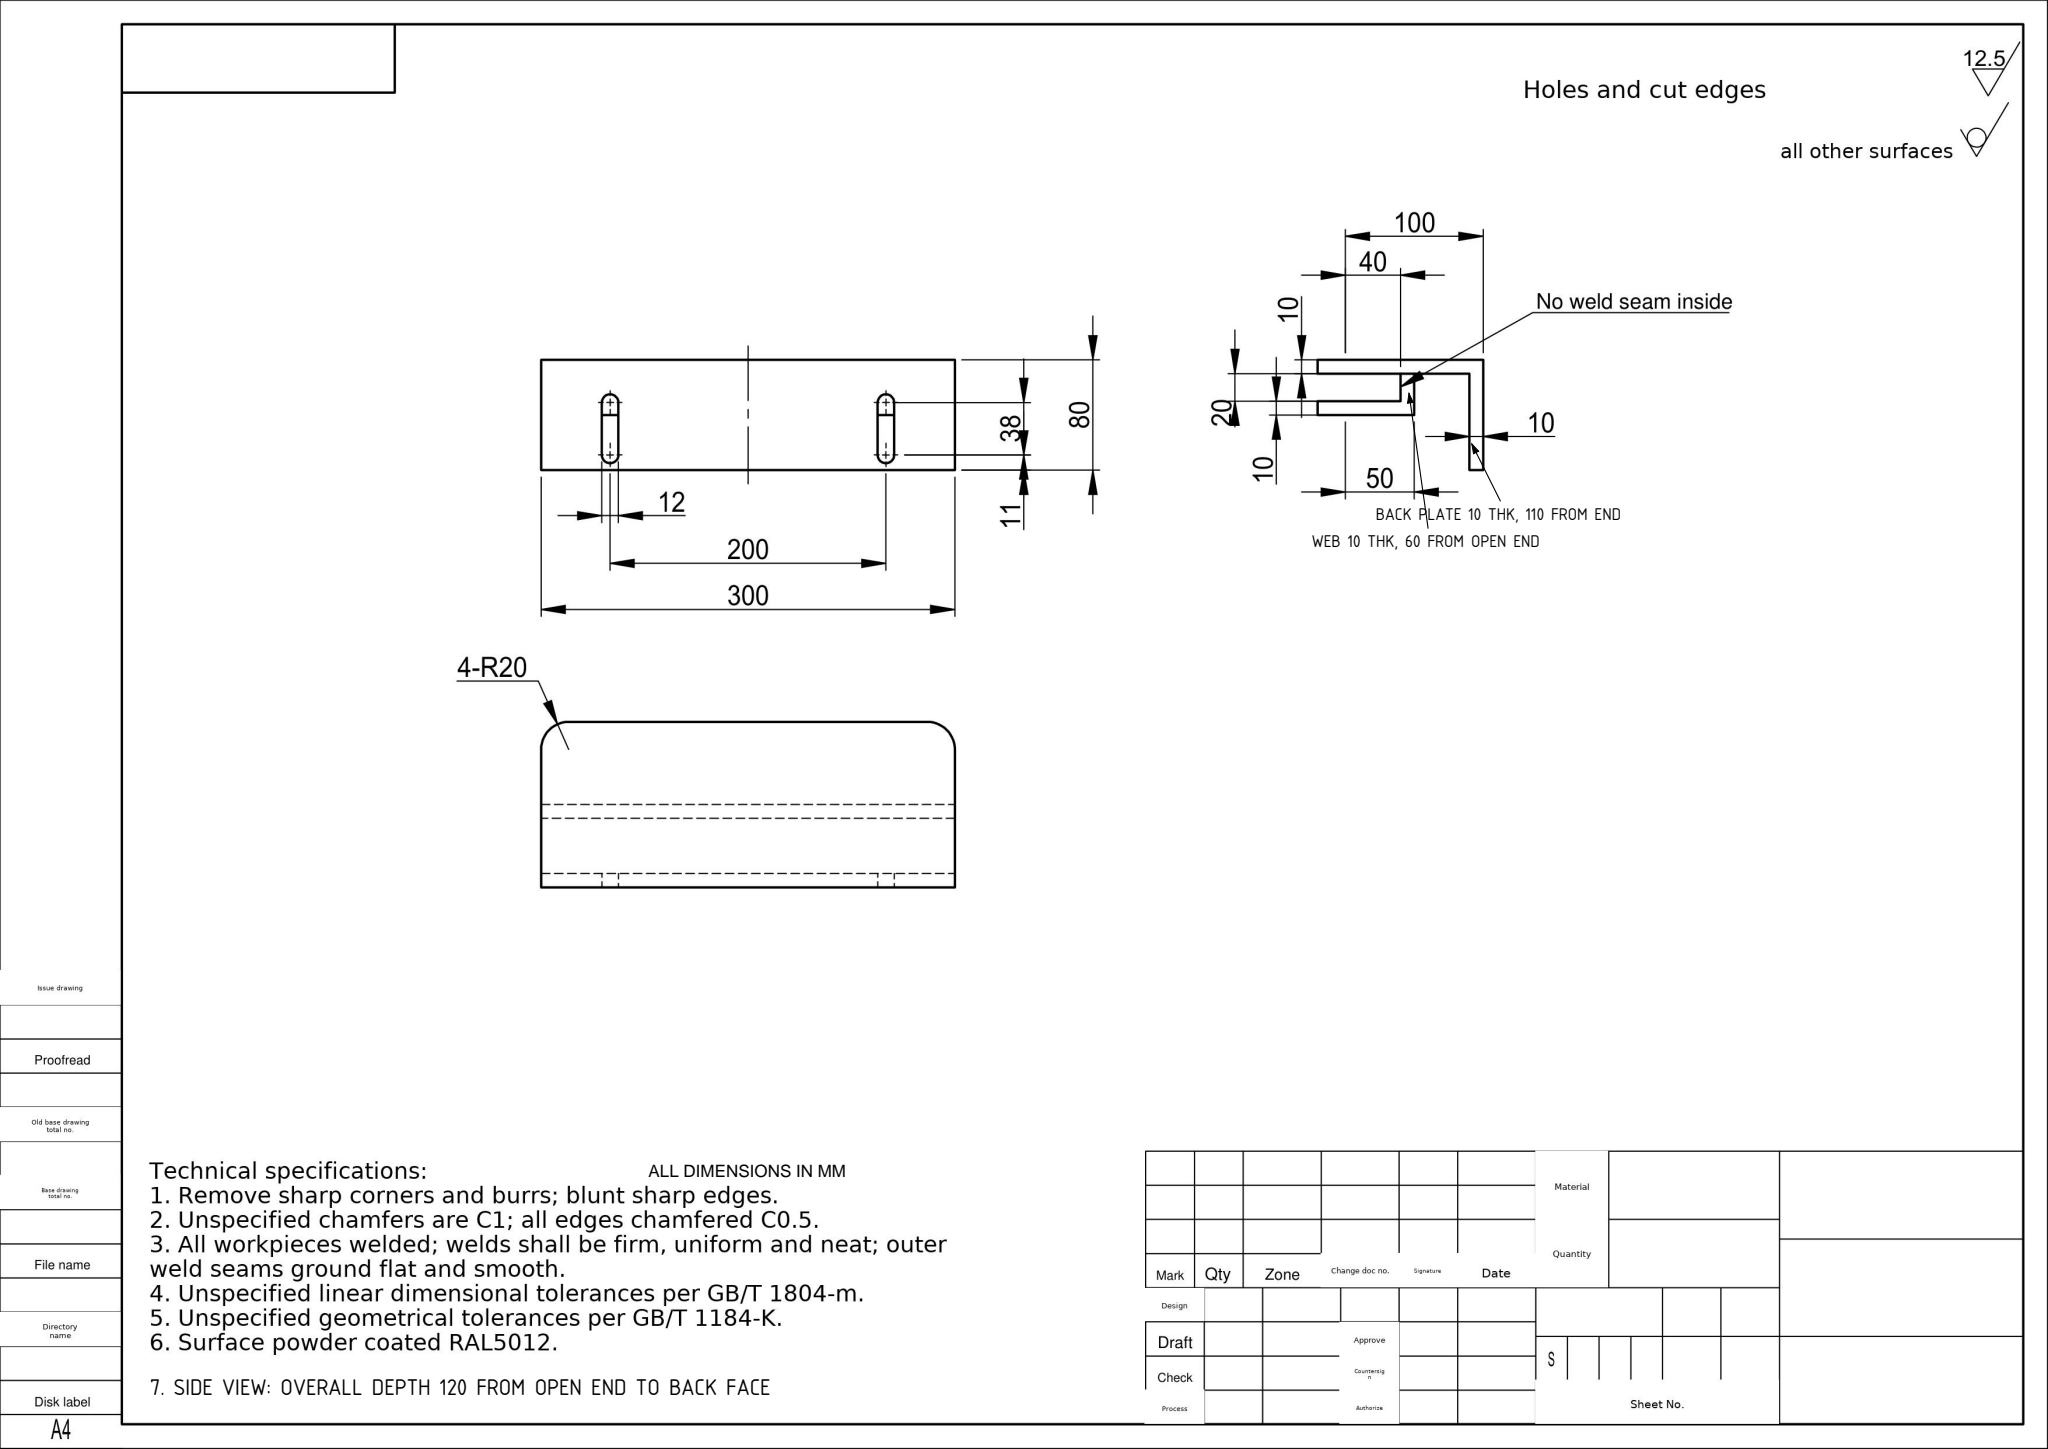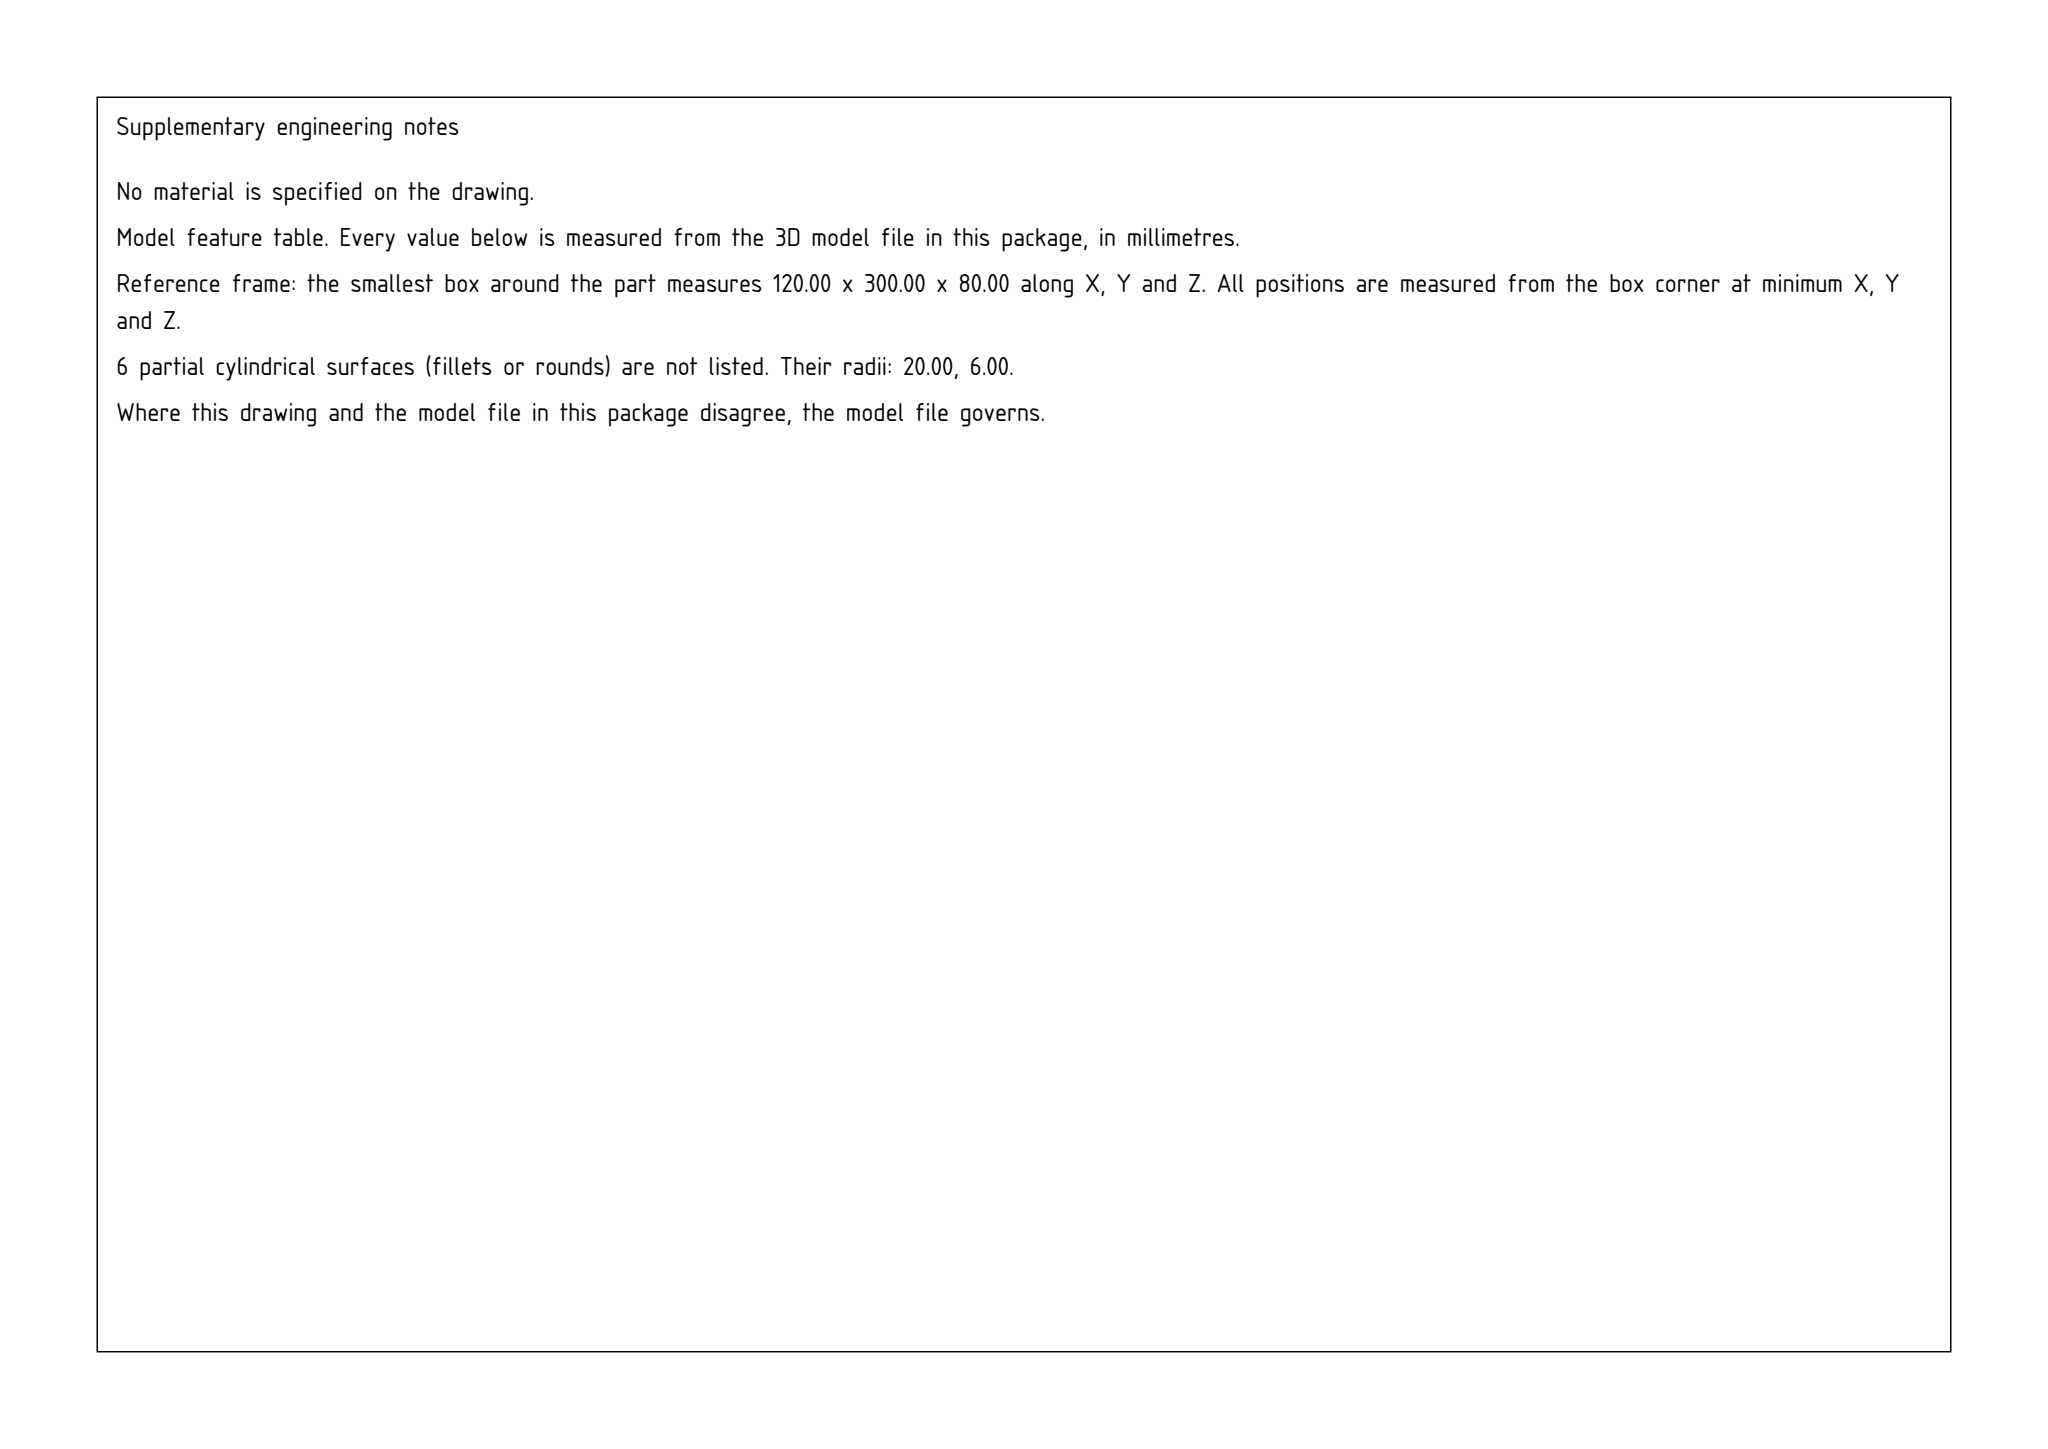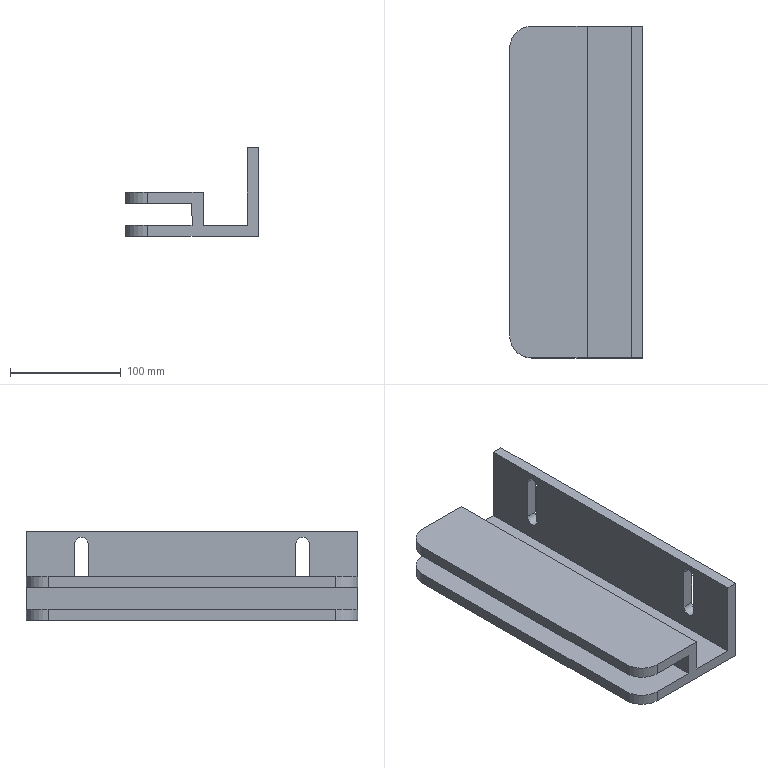Part | SolidWorks | mm | 1 solid | 28 faces | box 120 x 300 x 80 mm | volume 825184 mm3 | plane 18 | cylinder 10 | commonest cylinder face diameters 12 x6 40 x4
Drawing notes:
SIDE VIEW: OVERALL DEPTH 120 FROM OPEN END TO BACK FACE | from the solid: bbox_xyz x=120; planes x=0 (channel open end) and x=120 (back face)
BACK PLATE 10 THK: INNER FACE 110 FROM OPEN END | from the solid: plane x=110 (y 0-300, z 10-80) and plane x=120; 10 thk
WEB 10 THK: FACES 60 & 70 FROM OPEN END | from the solid: planes x=60 (z 10-30) and x=70 (z 10-40)
STEP:
#1=CARTESIAN_POINT('',(10.,-100.,-5.));
#2=VERTEX_POINT('',#1);
#3=CARTESIAN_POINT('',(10.,-94.,-11.));
#4=VERTEX_POINT('',#3);
#5=CARTESIAN_POINT('',(10.,-100.,-11.));
#6=DIRECTION('',(-1.,0.,0.));
#7=DIRECTION('',(0.,0.,1.));
#8=AXIS2_PLACEMENT_3D('',#5,#6,#7);
#9=CIRCLE('',#8,6.);
#10=EDGE_CURVE('',#2,#4,#9,.T.);
#11=ORIENTED_EDGE('',*,*,#10,.F.);
#12=CARTESIAN_POINT('',(-0.,-100.,-5.));
#13=VERTEX_POINT('',#12);
#14=CARTESIAN_POINT('',(0.,-100.,-5.));
#15=DIRECTION('',(-1.,0.,-0.));
#16=VECTOR('',#15,1000.);
#17=LINE('',#14,#16);
#18=EDGE_CURVE('',#2,#13,#17,.T.);
#19=ORIENTED_EDGE('',*,*,#18,.T.);
#20=CARTESIAN_POINT('',(0.,-94.,-11.));
#21=VERTEX_POINT('',#20);
#22=CARTESIAN_POINT('',(0.,-100.,-11.));
#23=DIRECTION('',(-1.,0.,-0.));
#24=DIRECTION('',(0.,0.,1.));
#25=AXIS2_PLACEMENT_3D('',#22,#23,#24);
#26=CIRCLE('',#25,6.);
#27=EDGE_CURVE('',#13,#21,#26,.T.);
#28=ORIENTED_EDGE('',*,*,#27,.T.);
#29=CARTESIAN_POINT('',(100.,-94.,-11.));
#30=DIRECTION('',(1.,-0.,0.));
#31=VECTOR('',#30,1000.);
#32=LINE('',#29,#31);
#33=EDGE_CURVE('',#21,#4,#32,.T.);
#34=ORIENTED_EDGE('',*,*,#33,.T.);
#35=EDGE_LOOP('',(#11,#19,#28,#34));
#36=FACE_OUTER_BOUND('',#35,.T.);
#37=CARTESIAN_POINT('',(0.,-100.,-11.));
#38=DIRECTION('',(-1.,0.,-0.));
#39=DIRECTION('',(0.,0.,1.));
#40=AXIS2_PLACEMENT_3D('',#37,#38,#39);
#41=CYLINDRICAL_SURFACE('',#40,6.);
#42=ADVANCED_FACE('',(#36),#41,.F.);
#43=CARTESIAN_POINT('',(10.,100.,-5.));
#44=VERTEX_POINT('',#43);
#45=CARTESIAN_POINT('',(10.,106.,-11.));
#46=VERTEX_POINT('',#45);
#47=CARTESIAN_POINT('',(10.,100.,-11.));
#48=DIRECTION('',(-1.,0.,0.));
#49=DIRECTION('',(0.,0.,1.));
#50=AXIS2_PLACEMENT_3D('',#47,#48,#49);
#51=CIRCLE('',#50,6.);
#52=EDGE_CURVE('',#44,#46,#51,.T.);
#53=ORIENTED_EDGE('',*,*,#52,.F.);
#54=CARTESIAN_POINT('',(-0.,100.,-5.));
#55=VERTEX_POINT('',#54);
#56=CARTESIAN_POINT('',(0.,100.,-5.));
#57=DIRECTION('',(-1.,0.,-0.));
#58=VECTOR('',#57,1000.);
#59=LINE('',#56,#58);
#60=EDGE_CURVE('',#44,#55,#59,.T.);
#61=ORIENTED_EDGE('',*,*,#60,.T.);
#62=CARTESIAN_POINT('',(0.,106.,-11.));
#63=VERTEX_POINT('',#62);
#64=CARTESIAN_POINT('',(0.,100.,-11.));
#65=DIRECTION('',(-1.,0.,-0.));
#66=DIRECTION('',(0.,0.,1.));
#67=AXIS2_PLACEMENT_3D('',#64,#65,#66);
#68=CIRCLE('',#67,6.);
#69=EDGE_CURVE('',#55,#63,#68,.T.);
#70=ORIENTED_EDGE('',*,*,#69,.T.);
#71=CARTESIAN_POINT('',(100.,106.,-11.));
#72=DIRECTION('',(1.,-0.,0.));
#73=VECTOR('',#72,1000.);
#74=LINE('',#71,#73);
#75=EDGE_CURVE('',#63,#46,#74,.T.);
#76=ORIENTED_EDGE('',*,*,#75,.T.);
#77=EDGE_LOOP('',(#53,#61,#70,#76));
#78=FACE_OUTER_BOUND('',#77,.T.);
#79=CARTESIAN_POINT('',(0.,100.,-11.));
#80=DIRECTION('',(-1.,0.,-0.));
#81=DIRECTION('',(0.,0.,1.));
#82=AXIS2_PLACEMENT_3D('',#79,#80,#81);
#83=CYLINDRICAL_SURFACE('',#82,6.);
#84=ADVANCED_FACE('',(#78),#83,.F.);
#85=CARTESIAN_POINT('',(-50.,150.,-50.));
#86=VERTEX_POINT('',#85);
#87=CARTESIAN_POINT('',(-50.,-150.,-50.));
#88=VERTEX_POINT('',#87);
#89=CARTESIAN_POINT('',(-50.,150.,-50.));
#90=DIRECTION('',(0.,-1.,0.));
#91=VECTOR('',#90,1000.);
#92=LINE('',#89,#91);
#93=EDGE_CURVE('',#86,#88,#92,.T.);
#94=ORIENTED_EDGE('',*,*,#93,.F.);
#95=CARTESIAN_POINT('',(-50.,150.,-70.));
#96=VERTEX_POINT('',#95);
#97=CARTESIAN_POINT('',(-50.,150.,-40.));
#98=DIRECTION('',(-0.,0.,-1.));
#99=VECTOR('',#98,1000.);
#100=LINE('',#97,#99);
#101=EDGE_CURVE('',#86,#96,#100,.T.);
#102=ORIENTED_EDGE('',*,*,#101,.T.);
#103=CARTESIAN_POINT('',(-50.,-150.,-70.));
#104=VERTEX_POINT('',#103);
#105=CARTESIAN_POINT('',(-50.,150.,-70.));
#106=DIRECTION('',(0.,-1.,0.));
#107=VECTOR('',#106,1000.);
#108=LINE('',#105,#107);
#109=EDGE_CURVE('',#96,#104,#108,.T.);
#110=ORIENTED_EDGE('',*,*,#109,.T.);
#111=CARTESIAN_POINT('',(-50.,-150.,-40.));
#112=DIRECTION('',(-0.,0.,-1.));
#113=VECTOR('',#112,1000.);
#114=LINE('',#111,#113);
#115=EDGE_CURVE('',#88,#104,#114,.T.);
#116=ORIENTED_EDGE('',*,*,#115,.F.);
#117=EDGE_LOOP('',(#94,#102,#110,#116));
#118=FACE_OUTER_BOUND('',#117,.T.);
#119=CARTESIAN_POINT('',(-50.,150.,-40.));
#120=DIRECTION('',(1.,0.,0.));
#121=DIRECTION('',(-0.,1.,0.));
#122=AXIS2_PLACEMENT_3D('',#119,#120,#121);
#123=PLANE('',#122);
#124=ADVANCED_FACE('',(#118),#123,.F.);
#125=CARTESIAN_POINT('',(-110.,130.,-70.));
#126=VERTEX_POINT('',#125);
#127=CARTESIAN_POINT('',(-110.,-130.,-70.));
#128=VERTEX_POINT('',#127);
#129=CARTESIAN_POINT('',(-110.,150.,-70.));
#130=DIRECTION('',(0.,-1.,0.));
#131=VECTOR('',#130,1000.);
#132=LINE('',#129,#131);
#133=EDGE_CURVE('',#126,#128,#132,.T.);
#134=ORIENTED_EDGE('',*,*,#133,.T.);
#135=CARTESIAN_POINT('',(-90.,-150.,-70.));
#136=VERTEX_POINT('',#135);
#137=CARTESIAN_POINT('',(-90.,-130.,-70.));
#138=DIRECTION('',(0.,0.,1.));
#139=DIRECTION('',(1.,0.,0.));
#140=AXIS2_PLACEMENT_3D('',#137,#138,#139);
#141=CIRCLE('',#140,20.);
#142=EDGE_CURVE('',#128,#136,#141,.T.);
#143=ORIENTED_EDGE('',*,*,#142,.T.);
#144=CARTESIAN_POINT('',(-110.,-150.,-70.));
#145=DIRECTION('',(-1.,0.,-0.));
#146=VECTOR('',#145,1000.);
#147=LINE('',#144,#146);
#148=EDGE_CURVE('',#104,#136,#147,.T.);
#149=ORIENTED_EDGE('',*,*,#148,.F.);
#150=ORIENTED_EDGE('',*,*,#109,.F.);
#151=CARTESIAN_POINT('',(-90.,150.,-70.));
#152=VERTEX_POINT('',#151);
#153=CARTESIAN_POINT('',(-110.,150.,-70.));
#154=DIRECTION('',(-1.,0.,-0.));
#155=VECTOR('',#154,1000.);
#156=LINE('',#153,#155);
#157=EDGE_CURVE('',#96,#152,#156,.T.);
#158=ORIENTED_EDGE('',*,*,#157,.T.);
#159=CARTESIAN_POINT('',(-90.,130.,-70.));
#160=DIRECTION('',(0.,0.,1.));
#161=DIRECTION('',(1.,0.,0.));
#162=AXIS2_PLACEMENT_3D('',#159,#160,#161);
#163=CIRCLE('',#162,20.);
#164=EDGE_CURVE('',#152,#126,#163,.T.);
#165=ORIENTED_EDGE('',*,*,#164,.T.);
#166=EDGE_LOOP('',(#134,#143,#149,#150,#158,#165));
#167=FACE_OUTER_BOUND('',#166,.T.);
#168=CARTESIAN_POINT('',(-110.,150.,-70.));
#169=DIRECTION('',(-0.,0.,1.));
#170=DIRECTION('',(1.,-0.,0.));
#171=AXIS2_PLACEMENT_3D('',#168,#169,#170);
#172=PLANE('',#171);
#173=ADVANCED_FACE('',(#167),#172,.T.);
#174=CARTESIAN_POINT('',(0.,150.,-70.));
#175=VERTEX_POINT('',#174);
#176=CARTESIAN_POINT('',(-40.,150.,-70.));
#177=VERTEX_POINT('',#176);
#178=CARTESIAN_POINT('',(-110.,150.,-70.));
#179=DIRECTION('',(-1.,0.,-0.));
#180=VECTOR('',#179,1000.);
#181=LINE('',#178,#180);
#182=EDGE_CURVE('',#175,#177,#181,.T.);
#183=ORIENTED_EDGE('',*,*,#182,.T.);
#184=CARTESIAN_POINT('',(-40.,-150.,-70.));
#185=VERTEX_POINT('',#184);
#186=CARTESIAN_POINT('',(-40.,150.,-70.));
#187=DIRECTION('',(-0.,1.,0.));
#188=VECTOR('',#187,1000.);
#189=LINE('',#186,#188);
#190=EDGE_CURVE('',#185,#177,#189,.T.);
#191=ORIENTED_EDGE('',*,*,#190,.F.);
#192=CARTESIAN_POINT('',(0.,-150.,-70.));
#193=VERTEX_POINT('',#192);
#194=CARTESIAN_POINT('',(-110.,-150.,-70.));
#195=DIRECTION('',(-1.,0.,-0.));
#196=VECTOR('',#195,1000.);
#197=LINE('',#194,#196);
#198=EDGE_CURVE('',#193,#185,#197,.T.);
#199=ORIENTED_EDGE('',*,*,#198,.F.);
#200=CARTESIAN_POINT('',(0.,150.,-70.));
#201=DIRECTION('',(0.,-1.,0.));
#202=VECTOR('',#201,1000.);
#203=LINE('',#200,#202);
#204=EDGE_CURVE('',#175,#193,#203,.T.);
#205=ORIENTED_EDGE('',*,*,#204,.F.);
#206=EDGE_LOOP('',(#183,#191,#199,#205));
#207=FACE_OUTER_BOUND('',#206,.T.);
#208=CARTESIAN_POINT('',(-110.,150.,-70.));
#209=DIRECTION('',(-0.,0.,1.));
#210=DIRECTION('',(1.,-0.,0.));
#211=AXIS2_PLACEMENT_3D('',#208,#209,#210);
#212=PLANE('',#211);
#213=ADVANCED_FACE('',(#207),#212,.T.);
#214=CARTESIAN_POINT('',(10.,-150.,-80.));
#215=VERTEX_POINT('',#214);
#216=CARTESIAN_POINT('',(-90.,-150.,-80.));
#217=VERTEX_POINT('',#216);
#218=CARTESIAN_POINT('',(-110.,-150.,-80.));
#219=DIRECTION('',(-1.,0.,-0.));
#220=VECTOR('',#219,1000.);
#221=LINE('',#218,#220);
#222=EDGE_CURVE('',#215,#217,#221,.T.);
#223=ORIENTED_EDGE('',*,*,#222,.T.);
#224=CARTESIAN_POINT('',(-110.,-130.,-80.));
#225=VERTEX_POINT('',#224);
#226=CARTESIAN_POINT('',(-90.,-130.,-80.));
#227=DIRECTION('',(-0.,0.,-1.));
#228=DIRECTION('',(1.,0.,0.));
#229=AXIS2_PLACEMENT_3D('',#226,#227,#228);
#230=CIRCLE('',#229,20.);
#231=EDGE_CURVE('',#217,#225,#230,.T.);
#232=ORIENTED_EDGE('',*,*,#231,.T.);
#233=CARTESIAN_POINT('',(-110.,130.,-80.));
#234=VERTEX_POINT('',#233);
#235=CARTESIAN_POINT('',(-110.,150.,-80.));
#236=DIRECTION('',(0.,-1.,0.));
#237=VECTOR('',#236,1000.);
#238=LINE('',#235,#237);
#239=EDGE_CURVE('',#234,#225,#238,.T.);
#240=ORIENTED_EDGE('',*,*,#239,.F.);
#241=CARTESIAN_POINT('',(-90.,150.,-80.));
#242=VERTEX_POINT('',#241);
#243=CARTESIAN_POINT('',(-90.,130.,-80.));
#244=DIRECTION('',(-0.,0.,-1.));
#245=DIRECTION('',(1.,0.,0.));
#246=AXIS2_PLACEMENT_3D('',#243,#244,#245);
#247=CIRCLE('',#246,20.);
#248=EDGE_CURVE('',#234,#242,#247,.T.);
#249=ORIENTED_EDGE('',*,*,#248,.T.);
#250=CARTESIAN_POINT('',(10.,150.,-80.));
#251=VERTEX_POINT('',#250);
#252=CARTESIAN_POINT('',(-110.,150.,-80.));
#253=DIRECTION('',(-1.,0.,-0.));
#254=VECTOR('',#253,1000.);
#255=LINE('',#252,#254);
#256=EDGE_CURVE('',#251,#242,#255,.T.);
#257=ORIENTED_EDGE('',*,*,#256,.F.);
#258=CARTESIAN_POINT('',(10.,150.,-80.));
#259=DIRECTION('',(0.,-1.,0.));
#260=VECTOR('',#259,1000.);
#261=LINE('',#258,#260);
#262=EDGE_CURVE('',#251,#215,#261,.T.);
#263=ORIENTED_EDGE('',*,*,#262,.T.);
#264=EDGE_LOOP('',(#223,#232,#240,#249,#257,#263));
#265=FACE_OUTER_BOUND('',#264,.T.);
#266=CARTESIAN_POINT('',(-110.,150.,-80.));
#267=DIRECTION('',(-0.,0.,1.));
#268=DIRECTION('',(1.,-0.,0.));
#269=AXIS2_PLACEMENT_3D('',#266,#267,#268);
#270=PLANE('',#269);
#271=ADVANCED_FACE('',(#265),#270,.F.);
#272=ORIENTED_EDGE('',*,*,#239,.T.);
#273=CARTESIAN_POINT('',(-110.,-130.,-70.));
#274=DIRECTION('',(-0.,-0.,1.));
#275=VECTOR('',#274,1000.);
#276=LINE('',#273,#275);
#277=EDGE_CURVE('',#225,#128,#276,.T.);
#278=ORIENTED_EDGE('',*,*,#277,.T.);
#279=ORIENTED_EDGE('',*,*,#133,.F.);
#280=CARTESIAN_POINT('',(-110.,130.,-70.));
#281=DIRECTION('',(0.,0.,-1.));
#282=VECTOR('',#281,1000.);
#283=LINE('',#280,#282);
#284=EDGE_CURVE('',#126,#234,#283,.T.);
#285=ORIENTED_EDGE('',*,*,#284,.T.);
#286=EDGE_LOOP('',(#272,#278,#279,#285));
#287=FACE_OUTER_BOUND('',#286,.T.);
#288=CARTESIAN_POINT('',(-110.,150.,-70.));
#289=DIRECTION('',(-1.,0.,0.));
#290=DIRECTION('',(0.,0.,1.));
#291=AXIS2_PLACEMENT_3D('',#288,#289,#290);
#292=PLANE('',#291);
#293=ADVANCED_FACE('',(#287),#292,.T.);
#294=CARTESIAN_POINT('',(0.,-106.,-11.));
#295=VERTEX_POINT('',#294);
#296=CARTESIAN_POINT('',(0.,-100.,-11.));
#297=DIRECTION('',(-1.,0.,-0.));
#298=DIRECTION('',(0.,0.,1.));
#299=AXIS2_PLACEMENT_3D('',#296,#297,#298);
#300=CIRCLE('',#299,6.);
#301=EDGE_CURVE('',#295,#13,#300,.T.);
#302=ORIENTED_EDGE('',*,*,#301,.F.);
#303=CARTESIAN_POINT('',(-0.,-106.,-49.));
#304=VERTEX_POINT('',#303);
#305=CARTESIAN_POINT('',(-0.,-106.,-49.));
#306=DIRECTION('',(0.,0.,1.));
#307=VECTOR('',#306,1000.);
#308=LINE('',#305,#307);
#309=EDGE_CURVE('',#304,#295,#308,.T.);
#310=ORIENTED_EDGE('',*,*,#309,.F.);
#311=CARTESIAN_POINT('',(-0.,-94.,-49.));
#312=VERTEX_POINT('',#311);
#313=CARTESIAN_POINT('',(-0.,-100.,-49.));
#314=DIRECTION('',(-1.,0.,-0.));
#315=DIRECTION('',(0.,0.,1.));
#316=AXIS2_PLACEMENT_3D('',#313,#314,#315);
#317=CIRCLE('',#316,6.);
#318=EDGE_CURVE('',#312,#304,#317,.T.);
#319=ORIENTED_EDGE('',*,*,#318,.F.);
#320=CARTESIAN_POINT('',(-0.,-94.,-49.));
#321=DIRECTION('',(0.,0.,1.));
#322=VECTOR('',#321,1000.);
#323=LINE('',#320,#322);
#324=EDGE_CURVE('',#312,#21,#323,.T.);
#325=ORIENTED_EDGE('',*,*,#324,.T.);
#326=ORIENTED_EDGE('',*,*,#27,.F.);
#327=EDGE_LOOP('',(#302,#310,#319,#325,#326));
#328=FACE_BOUND('',#327,.T.);
#329=CARTESIAN_POINT('',(0.,94.,-11.));
#330=VERTEX_POINT('',#329);
#331=CARTESIAN_POINT('',(0.,100.,-11.));
#332=DIRECTION('',(-1.,0.,-0.));
#333=DIRECTION('',(0.,0.,1.));
#334=AXIS2_PLACEMENT_3D('',#331,#332,#333);
#335=CIRCLE('',#334,6.);
#336=EDGE_CURVE('',#330,#55,#335,.T.);
#337=ORIENTED_EDGE('',*,*,#336,.F.);
#338=CARTESIAN_POINT('',(-0.,94.,-49.));
#339=VERTEX_POINT('',#338);
#340=CARTESIAN_POINT('',(-0.,94.,-49.));
#341=DIRECTION('',(0.,0.,1.));
#342=VECTOR('',#341,1000.);
#343=LINE('',#340,#342);
#344=EDGE_CURVE('',#339,#330,#343,.T.);
#345=ORIENTED_EDGE('',*,*,#344,.F.);
#346=CARTESIAN_POINT('',(-0.,106.,-49.));
#347=VERTEX_POINT('',#346);
#348=CARTESIAN_POINT('',(-0.,100.,-49.));
#349=DIRECTION('',(-1.,0.,-0.));
#350=DIRECTION('',(0.,0.,1.));
#351=AXIS2_PLACEMENT_3D('',#348,#349,#350);
#352=CIRCLE('',#351,6.);
#353=EDGE_CURVE('',#347,#339,#352,.T.);
#354=ORIENTED_EDGE('',*,*,#353,.F.);
#355=CARTESIAN_POINT('',(-0.,106.,-49.));
#356=DIRECTION('',(0.,0.,1.));
#357=VECTOR('',#356,1000.);
#358=LINE('',#355,#357);
#359=EDGE_CURVE('',#347,#63,#358,.T.);
#360=ORIENTED_EDGE('',*,*,#359,.T.);
#361=ORIENTED_EDGE('',*,*,#69,.F.);
#362=EDGE_LOOP('',(#337,#345,#354,#360,#361));
#363=FACE_BOUND('',#362,.T.);
#364=CARTESIAN_POINT('',(0.,-150.,0.));
#365=VERTEX_POINT('',#364);
#366=CARTESIAN_POINT('',(0.,-150.,-70.));
#367=DIRECTION('',(-0.,0.,-1.));
#368=VECTOR('',#367,1000.);
#369=LINE('',#366,#368);
#370=EDGE_CURVE('',#365,#193,#369,.T.);
#371=ORIENTED_EDGE('',*,*,#370,.F.);
#372=CARTESIAN_POINT('',(0.,150.,-0.));
#373=VERTEX_POINT('',#372);
#374=CARTESIAN_POINT('',(0.,150.,-0.));
#375=DIRECTION('',(0.,-1.,0.));
#376=VECTOR('',#375,1000.);
#377=LINE('',#374,#376);
#378=EDGE_CURVE('',#373,#365,#377,.T.);
#379=ORIENTED_EDGE('',*,*,#378,.F.);
#380=CARTESIAN_POINT('',(0.,150.,-70.));
#381=DIRECTION('',(-0.,0.,-1.));
#382=VECTOR('',#381,1000.);
#383=LINE('',#380,#382);
#384=EDGE_CURVE('',#373,#175,#383,.T.);
#385=ORIENTED_EDGE('',*,*,#384,.T.);
#386=ORIENTED_EDGE('',*,*,#204,.T.);
#387=EDGE_LOOP('',(#371,#379,#385,#386));
#388=FACE_OUTER_BOUND('',#387,.T.);
#389=CARTESIAN_POINT('',(0.,150.,-70.));
#390=DIRECTION('',(-1.,0.,0.));
#391=DIRECTION('',(0.,0.,1.));
#392=AXIS2_PLACEMENT_3D('',#389,#390,#391);
#393=PLANE('',#392);
#394=ADVANCED_FACE('',(#328,#363,#388),#393,.T.);
#395=CARTESIAN_POINT('',(10.,-150.,0.));
#396=VERTEX_POINT('',#395);
#397=CARTESIAN_POINT('',(10.,-150.,0.));
#398=DIRECTION('',(-1.,0.,-0.));
#399=VECTOR('',#398,1000.);
#400=LINE('',#397,#399);
#401=EDGE_CURVE('',#396,#365,#400,.T.);
#402=ORIENTED_EDGE('',*,*,#401,.F.);
#403=CARTESIAN_POINT('',(10.,150.,-0.));
#404=VERTEX_POINT('',#403);
#405=CARTESIAN_POINT('',(10.,150.,-0.));
#406=DIRECTION('',(0.,-1.,0.));
#407=VECTOR('',#406,1000.);
#408=LINE('',#405,#407);
#409=EDGE_CURVE('',#404,#396,#408,.T.);
#410=ORIENTED_EDGE('',*,*,#409,.F.);
#411=CARTESIAN_POINT('',(10.,150.,-0.));
#412=DIRECTION('',(-1.,0.,-0.));
#413=VECTOR('',#412,1000.);
#414=LINE('',#411,#413);
#415=EDGE_CURVE('',#404,#373,#414,.T.);
#416=ORIENTED_EDGE('',*,*,#415,.T.);
#417=ORIENTED_EDGE('',*,*,#378,.T.);
#418=EDGE_LOOP('',(#402,#410,#416,#417));
#419=FACE_OUTER_BOUND('',#418,.T.);
#420=CARTESIAN_POINT('',(10.,150.,-0.));
#421=DIRECTION('',(-0.,0.,1.));
#422=DIRECTION('',(1.,-0.,0.));
#423=AXIS2_PLACEMENT_3D('',#420,#421,#422);
#424=PLANE('',#423);
#425=ADVANCED_FACE('',(#419),#424,.T.);
#426=CARTESIAN_POINT('',(10.,-94.,-49.));
#427=VERTEX_POINT('',#426);
#428=CARTESIAN_POINT('',(10.,-94.,-70.));
#429=DIRECTION('',(0.,0.,1.));
#430=VECTOR('',#429,1000.);
#431=LINE('',#428,#430);
#432=EDGE_CURVE('',#427,#4,#431,.T.);
#433=ORIENTED_EDGE('',*,*,#432,.F.);
#434=CARTESIAN_POINT('',(10.,-106.,-49.));
#435=VERTEX_POINT('',#434);
#436=CARTESIAN_POINT('',(10.,-100.,-49.));
#437=DIRECTION('',(-1.,0.,0.));
#438=DIRECTION('',(0.,0.,1.));
#439=AXIS2_PLACEMENT_3D('',#436,#437,#438);
#440=CIRCLE('',#439,6.);
#441=EDGE_CURVE('',#427,#435,#440,.T.);
#442=ORIENTED_EDGE('',*,*,#441,.T.);
#443=CARTESIAN_POINT('',(10.,-106.,-11.));
#444=VERTEX_POINT('',#443);
#445=CARTESIAN_POINT('',(10.,-106.,-70.));
#446=DIRECTION('',(0.,0.,1.));
#447=VECTOR('',#446,1000.);
#448=LINE('',#445,#447);
#449=EDGE_CURVE('',#435,#444,#448,.T.);
#450=ORIENTED_EDGE('',*,*,#449,.T.);
#451=CARTESIAN_POINT('',(10.,-100.,-11.));
#452=DIRECTION('',(-1.,0.,0.));
#453=DIRECTION('',(0.,0.,1.));
#454=AXIS2_PLACEMENT_3D('',#451,#452,#453);
#455=CIRCLE('',#454,6.);
#456=EDGE_CURVE('',#444,#2,#455,.T.);
#457=ORIENTED_EDGE('',*,*,#456,.T.);
#458=ORIENTED_EDGE('',*,*,#10,.T.);
#459=EDGE_LOOP('',(#433,#442,#450,#457,#458));
#460=FACE_BOUND('',#459,.T.);
#461=CARTESIAN_POINT('',(10.,94.,-49.));
#462=VERTEX_POINT('',#461);
#463=CARTESIAN_POINT('',(10.,94.,-11.));
#464=VERTEX_POINT('',#463);
#465=CARTESIAN_POINT('',(10.,94.,-70.));
#466=DIRECTION('',(0.,0.,1.));
#467=VECTOR('',#466,1000.);
#468=LINE('',#465,#467);
#469=EDGE_CURVE('',#462,#464,#468,.T.);
#470=ORIENTED_EDGE('',*,*,#469,.T.);
#471=CARTESIAN_POINT('',(10.,100.,-11.));
#472=DIRECTION('',(-1.,0.,0.));
#473=DIRECTION('',(0.,0.,1.));
#474=AXIS2_PLACEMENT_3D('',#471,#472,#473);
#475=CIRCLE('',#474,6.);
#476=EDGE_CURVE('',#464,#44,#475,.T.);
#477=ORIENTED_EDGE('',*,*,#476,.T.);
#478=ORIENTED_EDGE('',*,*,#52,.T.);
#479=CARTESIAN_POINT('',(10.,106.,-49.));
#480=VERTEX_POINT('',#479);
#481=CARTESIAN_POINT('',(10.,106.,-70.));
#482=DIRECTION('',(0.,0.,1.));
#483=VECTOR('',#482,1000.);
#484=LINE('',#481,#483);
#485=EDGE_CURVE('',#480,#46,#484,.T.);
#486=ORIENTED_EDGE('',*,*,#485,.F.);
#487=CARTESIAN_POINT('',(10.,100.,-49.));
#488=DIRECTION('',(-1.,0.,0.));
#489=DIRECTION('',(0.,0.,1.));
#490=AXIS2_PLACEMENT_3D('',#487,#488,#489);
#491=CIRCLE('',#490,6.);
#492=EDGE_CURVE('',#480,#462,#491,.T.);
#493=ORIENTED_EDGE('',*,*,#492,.T.);
#494=EDGE_LOOP('',(#470,#477,#478,#486,#493));
#495=FACE_BOUND('',#494,.T.);
#496=CARTESIAN_POINT('',(10.,-150.,-70.));
#497=DIRECTION('',(-0.,0.,-1.));
#498=VECTOR('',#497,1000.);
#499=LINE('',#496,#498);
#500=EDGE_CURVE('',#396,#215,#499,.T.);
#501=ORIENTED_EDGE('',*,*,#500,.T.);
#502=ORIENTED_EDGE('',*,*,#262,.F.);
#503=CARTESIAN_POINT('',(10.,150.,-70.));
#504=DIRECTION('',(-0.,0.,-1.));
#505=VECTOR('',#504,1000.);
#506=LINE('',#503,#505);
#507=EDGE_CURVE('',#404,#251,#506,.T.);
#508=ORIENTED_EDGE('',*,*,#507,.F.);
#509=ORIENTED_EDGE('',*,*,#409,.T.);
#510=EDGE_LOOP('',(#501,#502,#508,#509));
#511=FACE_OUTER_BOUND('',#510,.T.);
#512=CARTESIAN_POINT('',(10.,150.,-70.));
#513=DIRECTION('',(-1.,0.,0.));
#514=DIRECTION('',(0.,0.,1.));
#515=AXIS2_PLACEMENT_3D('',#512,#513,#514);
#516=PLANE('',#515);
#517=ADVANCED_FACE('',(#460,#495,#511),#516,.F.);
#518=CARTESIAN_POINT('',(-90.,150.,-50.));
#519=VERTEX_POINT('',#518);
#520=CARTESIAN_POINT('',(-410.167,150.,-50.));
#521=DIRECTION('',(1.,0.,0.));
#522=VECTOR('',#521,1000.);
#523=LINE('',#520,#522);
#524=EDGE_CURVE('',#519,#86,#523,.T.);
#525=ORIENTED_EDGE('',*,*,#524,.F.);
#526=CARTESIAN_POINT('',(-90.,150.,-40.));
#527=VERTEX_POINT('',#526);
#528=CARTESIAN_POINT('',(-90.,150.,-0.));
#529=DIRECTION('',(-0.,-0.,1.));
#530=VECTOR('',#529,1000.);
#531=LINE('',#528,#530);
#532=EDGE_CURVE('',#519,#527,#531,.T.);
#533=ORIENTED_EDGE('',*,*,#532,.T.);
#534=CARTESIAN_POINT('',(-40.,150.,-40.));
#535=VERTEX_POINT('',#534);
#536=CARTESIAN_POINT('',(-50.,150.,-40.));
#537=DIRECTION('',(-1.,0.,-0.));
#538=VECTOR('',#537,1000.);
#539=LINE('',#536,#538);
#540=EDGE_CURVE('',#535,#527,#539,.T.);
#541=ORIENTED_EDGE('',*,*,#540,.F.);
#542=CARTESIAN_POINT('',(-40.,150.,-40.));
#543=DIRECTION('',(-0.,0.,-1.));
#544=VECTOR('',#543,1000.);
#545=LINE('',#542,#544);
#546=EDGE_CURVE('',#535,#177,#545,.T.);
#547=ORIENTED_EDGE('',*,*,#546,.T.);
#548=ORIENTED_EDGE('',*,*,#182,.F.);
#549=ORIENTED_EDGE('',*,*,#384,.F.);
#550=ORIENTED_EDGE('',*,*,#415,.F.);
#551=ORIENTED_EDGE('',*,*,#507,.T.);
#552=ORIENTED_EDGE('',*,*,#256,.T.);
#553=CARTESIAN_POINT('',(-90.,150.,-0.));
#554=DIRECTION('',(-0.,-0.,1.));
#555=VECTOR('',#554,1000.);
#556=LINE('',#553,#555);
#557=EDGE_CURVE('',#242,#152,#556,.T.);
#558=ORIENTED_EDGE('',*,*,#557,.T.);
#559=ORIENTED_EDGE('',*,*,#157,.F.);
#560=ORIENTED_EDGE('',*,*,#101,.F.);
#561=EDGE_LOOP('',(#525,#533,#541,#547,#548,#549,#550,#551,#552,#558,#559,#560));
#562=FACE_OUTER_BOUND('',#561,.T.);
#563=CARTESIAN_POINT('',(0.,150.,-0.));
#564=DIRECTION('',(0.,1.,0.));
#565=DIRECTION('',(1.,-0.,0.));
#566=AXIS2_PLACEMENT_3D('',#563,#564,#565);
#567=PLANE('',#566);
#568=ADVANCED_FACE('',(#562),#567,.T.);
#569=CARTESIAN_POINT('',(-90.,-150.,-40.));
#570=VERTEX_POINT('',#569);
#571=CARTESIAN_POINT('',(-40.,-150.,-40.));
#572=VERTEX_POINT('',#571);
#573=CARTESIAN_POINT('',(-50.,-150.,-40.));
#574=DIRECTION('',(1.,-0.,0.));
#575=VECTOR('',#574,1000.);
#576=LINE('',#573,#575);
#577=EDGE_CURVE('',#570,#572,#576,.T.);
#578=ORIENTED_EDGE('',*,*,#577,.F.);
#579=CARTESIAN_POINT('',(-90.,-150.,-50.));
#580=VERTEX_POINT('',#579);
#581=CARTESIAN_POINT('',(-90.,-150.,-50.));
#582=DIRECTION('',(0.,0.,-1.));
#583=VECTOR('',#582,1000.);
#584=LINE('',#581,#583);
#585=EDGE_CURVE('',#570,#580,#584,.T.);
#586=ORIENTED_EDGE('',*,*,#585,.T.);
#587=CARTESIAN_POINT('',(-410.167,-150.,-50.));
#588=DIRECTION('',(1.,0.,0.));
#589=VECTOR('',#588,1000.);
#590=LINE('',#587,#589);
#591=EDGE_CURVE('',#580,#88,#590,.T.);
#592=ORIENTED_EDGE('',*,*,#591,.T.);
#593=ORIENTED_EDGE('',*,*,#115,.T.);
#594=ORIENTED_EDGE('',*,*,#148,.T.);
#595=CARTESIAN_POINT('',(-90.,-150.,-80.));
#596=DIRECTION('',(0.,0.,-1.));
#597=VECTOR('',#596,1000.);
#598=LINE('',#595,#597);
#599=EDGE_CURVE('',#136,#217,#598,.T.);
#600=ORIENTED_EDGE('',*,*,#599,.T.);
#601=ORIENTED_EDGE('',*,*,#222,.F.);
#602=ORIENTED_EDGE('',*,*,#500,.F.);
#603=ORIENTED_EDGE('',*,*,#401,.T.);
#604=ORIENTED_EDGE('',*,*,#370,.T.);
#605=ORIENTED_EDGE('',*,*,#198,.T.);
#606=CARTESIAN_POINT('',(-40.,-150.,-40.));
#607=DIRECTION('',(-0.,0.,-1.));
#608=VECTOR('',#607,1000.);
#609=LINE('',#606,#608);
#610=EDGE_CURVE('',#572,#185,#609,.T.);
#611=ORIENTED_EDGE('',*,*,#610,.F.);
#612=EDGE_LOOP('',(#578,#586,#592,#593,#594,#600,#601,#602,#603,#604,#605,#611));
#613=FACE_OUTER_BOUND('',#612,.T.);
#614=CARTESIAN_POINT('',(0.,-150.,0.));
#615=DIRECTION('',(0.,1.,0.));
#616=DIRECTION('',(1.,-0.,0.));
#617=AXIS2_PLACEMENT_3D('',#614,#615,#616);
#618=PLANE('',#617);
#619=ADVANCED_FACE('',(#613),#618,.F.);
#620=ORIENTED_EDGE('',*,*,#190,.T.);
#621=ORIENTED_EDGE('',*,*,#546,.F.);
#622=CARTESIAN_POINT('',(-40.,150.,-40.));
#623=DIRECTION('',(-0.,1.,0.));
#624=VECTOR('',#623,1000.);
#625=LINE('',#622,#624);
#626=EDGE_CURVE('',#572,#535,#625,.T.);
#627=ORIENTED_EDGE('',*,*,#626,.F.);
#628=ORIENTED_EDGE('',*,*,#610,.T.);
#629=EDGE_LOOP('',(#620,#621,#627,#628));
#630=FACE_OUTER_BOUND('',#629,.T.);
#631=CARTESIAN_POINT('',(-40.,150.,-40.));
#632=DIRECTION('',(-1.,-0.,-0.));
#633=DIRECTION('',(0.,-1.,0.));
#634=AXIS2_PLACEMENT_3D('',#631,#632,#633);
#635=PLANE('',#634);
#636=ADVANCED_FACE('',(#630),#635,.F.);
#637=CARTESIAN_POINT('',(-110.,-130.,-40.));
#638=VERTEX_POINT('',#637);
#639=CARTESIAN_POINT('',(-110.,130.,-40.));
#640=VERTEX_POINT('',#639);
#641=CARTESIAN_POINT('',(-110.,150.,-40.));
#642=DIRECTION('',(-0.,1.,-0.));
#643=VECTOR('',#642,1000.);
#644=LINE('',#641,#643);
#645=EDGE_CURVE('',#638,#640,#644,.T.);
#646=ORIENTED_EDGE('',*,*,#645,.F.);
#647=CARTESIAN_POINT('',(-90.,-130.,-40.));
#648=DIRECTION('',(0.,0.,1.));
#649=DIRECTION('',(1.,0.,0.));
#650=AXIS2_PLACEMENT_3D('',#647,#648,#649);
#651=CIRCLE('',#650,20.);
#652=EDGE_CURVE('',#638,#570,#651,.T.);
#653=ORIENTED_EDGE('',*,*,#652,.T.);
#654=ORIENTED_EDGE('',*,*,#577,.T.);
#655=ORIENTED_EDGE('',*,*,#626,.T.);
#656=ORIENTED_EDGE('',*,*,#540,.T.);
#657=CARTESIAN_POINT('',(-90.,130.,-40.));
#658=DIRECTION('',(0.,0.,1.));
#659=DIRECTION('',(1.,0.,0.));
#660=AXIS2_PLACEMENT_3D('',#657,#658,#659);
#661=CIRCLE('',#660,20.);
#662=EDGE_CURVE('',#527,#640,#661,.T.);
#663=ORIENTED_EDGE('',*,*,#662,.T.);
#664=EDGE_LOOP('',(#646,#653,#654,#655,#656,#663));
#665=FACE_OUTER_BOUND('',#664,.T.);
#666=CARTESIAN_POINT('',(-0.,0.,-40.));
#667=DIRECTION('',(-0.,0.,1.));
#668=DIRECTION('',(1.,-0.,0.));
#669=AXIS2_PLACEMENT_3D('',#666,#667,#668);
#670=PLANE('',#669);
#671=ADVANCED_FACE('',(#665),#670,.T.);
#672=ORIENTED_EDGE('',*,*,#591,.F.);
#673=CARTESIAN_POINT('',(-110.,-130.,-50.));
#674=VERTEX_POINT('',#673);
#675=CARTESIAN_POINT('',(-90.,-130.,-50.));
#676=DIRECTION('',(-0.,-0.,-1.));
#677=DIRECTION('',(0.,-1.,0.));
#678=AXIS2_PLACEMENT_3D('',#675,#676,#677);
#679=CIRCLE('',#678,20.);
#680=EDGE_CURVE('',#580,#674,#679,.T.);
#681=ORIENTED_EDGE('',*,*,#680,.T.);
#682=CARTESIAN_POINT('',(-110.,130.,-50.));
#683=VERTEX_POINT('',#682);
#684=CARTESIAN_POINT('',(-110.,150.,-50.));
#685=DIRECTION('',(0.,-1.,0.));
#686=VECTOR('',#685,1000.);
#687=LINE('',#684,#686);
#688=EDGE_CURVE('',#683,#674,#687,.T.);
#689=ORIENTED_EDGE('',*,*,#688,.F.);
#690=CARTESIAN_POINT('',(-90.,130.,-50.));
#691=DIRECTION('',(-0.,-0.,-1.));
#692=DIRECTION('',(0.,-1.,0.));
#693=AXIS2_PLACEMENT_3D('',#690,#691,#692);
#694=CIRCLE('',#693,20.);
#695=EDGE_CURVE('',#683,#519,#694,.T.);
#696=ORIENTED_EDGE('',*,*,#695,.T.);
#697=ORIENTED_EDGE('',*,*,#524,.T.);
#698=ORIENTED_EDGE('',*,*,#93,.T.);
#699=EDGE_LOOP('',(#672,#681,#689,#696,#697,#698));
#700=FACE_OUTER_BOUND('',#699,.T.);
#701=CARTESIAN_POINT('',(-410.167,150.,-50.));
#702=DIRECTION('',(0.,0.,1.));
#703=DIRECTION('',(0.,-1.,0.));
#704=AXIS2_PLACEMENT_3D('',#701,#702,#703);
#705=PLANE('',#704);
#706=ADVANCED_FACE('',(#700),#705,.F.);
#707=ORIENTED_EDGE('',*,*,#688,.T.);
#708=CARTESIAN_POINT('',(-110.,-130.,-40.));
#709=DIRECTION('',(-0.,-0.,1.));
#710=VECTOR('',#709,1000.);
#711=LINE('',#708,#710);
#712=EDGE_CURVE('',#674,#638,#711,.T.);
#713=ORIENTED_EDGE('',*,*,#712,.T.);
#714=ORIENTED_EDGE('',*,*,#645,.T.);
#715=CARTESIAN_POINT('',(-110.,130.,-70.));
#716=DIRECTION('',(0.,0.,-1.));
#717=VECTOR('',#716,1000.);
#718=LINE('',#715,#717);
#719=EDGE_CURVE('',#640,#683,#718,.T.);
#720=ORIENTED_EDGE('',*,*,#719,.T.);
#721=EDGE_LOOP('',(#707,#713,#714,#720));
#722=FACE_OUTER_BOUND('',#721,.T.);
#723=CARTESIAN_POINT('',(-110.,150.,-70.));
#724=DIRECTION('',(-1.,0.,0.));
#725=DIRECTION('',(0.,0.,1.));
#726=AXIS2_PLACEMENT_3D('',#723,#724,#725);
#727=PLANE('',#726);
#728=ADVANCED_FACE('',(#722),#727,.T.);
#729=ORIENTED_EDGE('',*,*,#60,.F.);
#730=ORIENTED_EDGE('',*,*,#476,.F.);
#731=CARTESIAN_POINT('',(0.,94.,-11.));
#732=DIRECTION('',(1.,-0.,0.));
#733=VECTOR('',#732,1000.);
#734=LINE('',#731,#733);
#735=EDGE_CURVE('',#330,#464,#734,.T.);
#736=ORIENTED_EDGE('',*,*,#735,.F.);
#737=ORIENTED_EDGE('',*,*,#336,.T.);
#738=EDGE_LOOP('',(#729,#730,#736,#737));
#739=FACE_OUTER_BOUND('',#738,.T.);
#740=CARTESIAN_POINT('',(0.,100.,-11.));
#741=DIRECTION('',(-1.,0.,-0.));
#742=DIRECTION('',(0.,0.,1.));
#743=AXIS2_PLACEMENT_3D('',#740,#741,#742);
#744=CYLINDRICAL_SURFACE('',#743,6.);
#745=ADVANCED_FACE('',(#739),#744,.F.);
#746=CARTESIAN_POINT('',(100.,106.,-49.));
#747=DIRECTION('',(1.,-0.,0.));
#748=VECTOR('',#747,1000.);
#749=LINE('',#746,#748);
#750=EDGE_CURVE('',#347,#480,#749,.T.);
#751=ORIENTED_EDGE('',*,*,#750,.F.);
#752=ORIENTED_EDGE('',*,*,#353,.T.);
#753=CARTESIAN_POINT('',(-0.,94.,-49.));
#754=DIRECTION('',(-1.,0.,-0.));
#755=VECTOR('',#754,1000.);
#756=LINE('',#753,#755);
#757=EDGE_CURVE('',#462,#339,#756,.T.);
#758=ORIENTED_EDGE('',*,*,#757,.F.);
#759=ORIENTED_EDGE('',*,*,#492,.F.);
#760=EDGE_LOOP('',(#751,#752,#758,#759));
#761=FACE_OUTER_BOUND('',#760,.T.);
#762=CARTESIAN_POINT('',(-0.,100.,-49.));
#763=DIRECTION('',(-1.,0.,-0.));
#764=DIRECTION('',(0.,0.,1.));
#765=AXIS2_PLACEMENT_3D('',#762,#763,#764);
#766=CYLINDRICAL_SURFACE('',#765,6.);
#767=ADVANCED_FACE('',(#761),#766,.F.);
#768=ORIENTED_EDGE('',*,*,#757,.T.);
#769=ORIENTED_EDGE('',*,*,#344,.T.);
#770=ORIENTED_EDGE('',*,*,#735,.T.);
#771=ORIENTED_EDGE('',*,*,#469,.F.);
#772=EDGE_LOOP('',(#768,#769,#770,#771));
#773=FACE_OUTER_BOUND('',#772,.T.);
#774=CARTESIAN_POINT('',(-0.,94.,-49.));
#775=DIRECTION('',(0.,-1.,-0.));
#776=DIRECTION('',(-0.,0.,-1.));
#777=AXIS2_PLACEMENT_3D('',#774,#775,#776);
#778=PLANE('',#777);
#779=ADVANCED_FACE('',(#773),#778,.F.);
#780=ORIENTED_EDGE('',*,*,#485,.T.);
#781=ORIENTED_EDGE('',*,*,#75,.F.);
#782=ORIENTED_EDGE('',*,*,#359,.F.);
#783=ORIENTED_EDGE('',*,*,#750,.T.);
#784=EDGE_LOOP('',(#780,#781,#782,#783));
#785=FACE_OUTER_BOUND('',#784,.T.);
#786=CARTESIAN_POINT('',(100.,106.,-49.));
#787=DIRECTION('',(-0.,-1.,-0.));
#788=DIRECTION('',(1.,-0.,0.));
#789=AXIS2_PLACEMENT_3D('',#786,#787,#788);
#790=PLANE('',#789);
#791=ADVANCED_FACE('',(#785),#790,.T.);
#792=CARTESIAN_POINT('',(100.,-94.,-49.));
#793=DIRECTION('',(1.,-0.,0.));
#794=VECTOR('',#793,1000.);
#795=LINE('',#792,#794);
#796=EDGE_CURVE('',#312,#427,#795,.T.);
#797=ORIENTED_EDGE('',*,*,#796,.F.);
#798=ORIENTED_EDGE('',*,*,#318,.T.);
#799=CARTESIAN_POINT('',(-0.,-106.,-49.));
#800=DIRECTION('',(-1.,0.,-0.));
#801=VECTOR('',#800,1000.);
#802=LINE('',#799,#801);
#803=EDGE_CURVE('',#435,#304,#802,.T.);
#804=ORIENTED_EDGE('',*,*,#803,.F.);
#805=ORIENTED_EDGE('',*,*,#441,.F.);
#806=EDGE_LOOP('',(#797,#798,#804,#805));
#807=FACE_OUTER_BOUND('',#806,.T.);
#808=CARTESIAN_POINT('',(-0.,-100.,-49.));
#809=DIRECTION('',(-1.,0.,-0.));
#810=DIRECTION('',(0.,0.,1.));
#811=AXIS2_PLACEMENT_3D('',#808,#809,#810);
#812=CYLINDRICAL_SURFACE('',#811,6.);
#813=ADVANCED_FACE('',(#807),#812,.F.);
#814=ORIENTED_EDGE('',*,*,#432,.T.);
#815=ORIENTED_EDGE('',*,*,#33,.F.);
#816=ORIENTED_EDGE('',*,*,#324,.F.);
#817=ORIENTED_EDGE('',*,*,#796,.T.);
#818=EDGE_LOOP('',(#814,#815,#816,#817));
#819=FACE_OUTER_BOUND('',#818,.T.);
#820=CARTESIAN_POINT('',(100.,-94.,-49.));
#821=DIRECTION('',(-0.,-1.,-0.));
#822=DIRECTION('',(1.,-0.,0.));
#823=AXIS2_PLACEMENT_3D('',#820,#821,#822);
#824=PLANE('',#823);
#825=ADVANCED_FACE('',(#819),#824,.T.);
#826=ORIENTED_EDGE('',*,*,#18,.F.);
#827=ORIENTED_EDGE('',*,*,#456,.F.);
#828=CARTESIAN_POINT('',(0.,-106.,-11.));
#829=DIRECTION('',(1.,-0.,0.));
#830=VECTOR('',#829,1000.);
#831=LINE('',#828,#830);
#832=EDGE_CURVE('',#295,#444,#831,.T.);
#833=ORIENTED_EDGE('',*,*,#832,.F.);
#834=ORIENTED_EDGE('',*,*,#301,.T.);
#835=EDGE_LOOP('',(#826,#827,#833,#834));
#836=FACE_OUTER_BOUND('',#835,.T.);
#837=CARTESIAN_POINT('',(0.,-100.,-11.));
#838=DIRECTION('',(-1.,0.,-0.));
#839=DIRECTION('',(0.,0.,1.));
#840=AXIS2_PLACEMENT_3D('',#837,#838,#839);
#841=CYLINDRICAL_SURFACE('',#840,6.);
#842=ADVANCED_FACE('',(#836),#841,.F.);
#843=ORIENTED_EDGE('',*,*,#803,.T.);
#844=ORIENTED_EDGE('',*,*,#309,.T.);
#845=ORIENTED_EDGE('',*,*,#832,.T.);
#846=ORIENTED_EDGE('',*,*,#449,.F.);
#847=EDGE_LOOP('',(#843,#844,#845,#846));
#848=FACE_OUTER_BOUND('',#847,.T.);
#849=CARTESIAN_POINT('',(-0.,-106.,-49.));
#850=DIRECTION('',(0.,-1.,-0.));
#851=DIRECTION('',(-0.,0.,-1.));
#852=AXIS2_PLACEMENT_3D('',#849,#850,#851);
#853=PLANE('',#852);
#854=ADVANCED_FACE('',(#848),#853,.F.);
#855=ORIENTED_EDGE('',*,*,#680,.F.);
#856=ORIENTED_EDGE('',*,*,#585,.F.);
#857=ORIENTED_EDGE('',*,*,#652,.F.);
#858=ORIENTED_EDGE('',*,*,#712,.F.);
#859=EDGE_LOOP('',(#855,#856,#857,#858));
#860=FACE_OUTER_BOUND('',#859,.T.);
#861=CARTESIAN_POINT('',(-90.,-130.,-70.));
#862=DIRECTION('',(0.,0.,-1.));
#863=DIRECTION('',(-1.,0.,0.));
#864=AXIS2_PLACEMENT_3D('',#861,#862,#863);
#865=CYLINDRICAL_SURFACE('',#864,20.);
#866=ADVANCED_FACE('',(#860),#865,.T.);
#867=ORIENTED_EDGE('',*,*,#142,.F.);
#868=ORIENTED_EDGE('',*,*,#277,.F.);
#869=ORIENTED_EDGE('',*,*,#231,.F.);
#870=ORIENTED_EDGE('',*,*,#599,.F.);
#871=EDGE_LOOP('',(#867,#868,#869,#870));
#872=FACE_OUTER_BOUND('',#871,.T.);
#873=CARTESIAN_POINT('',(-90.,-130.,0.));
#874=DIRECTION('',(-0.,-0.,1.));
#875=DIRECTION('',(1.,0.,0.));
#876=AXIS2_PLACEMENT_3D('',#873,#874,#875);
#877=CYLINDRICAL_SURFACE('',#876,20.);
#878=ADVANCED_FACE('',(#872),#877,.T.);
#879=ORIENTED_EDGE('',*,*,#662,.F.);
#880=ORIENTED_EDGE('',*,*,#532,.F.);
#881=ORIENTED_EDGE('',*,*,#695,.F.);
#882=ORIENTED_EDGE('',*,*,#719,.F.);
#883=EDGE_LOOP('',(#879,#880,#881,#882));
#884=FACE_OUTER_BOUND('',#883,.T.);
#885=CARTESIAN_POINT('',(-90.,130.,-70.));
#886=DIRECTION('',(0.,0.,-1.));
#887=DIRECTION('',(-1.,0.,0.));
#888=AXIS2_PLACEMENT_3D('',#885,#886,#887);
#889=CYLINDRICAL_SURFACE('',#888,20.);
#890=ADVANCED_FACE('',(#884),#889,.T.);
#891=ORIENTED_EDGE('',*,*,#164,.F.);
#892=ORIENTED_EDGE('',*,*,#557,.F.);
#893=ORIENTED_EDGE('',*,*,#248,.F.);
#894=ORIENTED_EDGE('',*,*,#284,.F.);
#895=EDGE_LOOP('',(#891,#892,#893,#894));
#896=FACE_OUTER_BOUND('',#895,.T.);
#897=CARTESIAN_POINT('',(-90.,130.,-70.));
#898=DIRECTION('',(0.,0.,-1.));
#899=DIRECTION('',(-1.,0.,0.));
#900=AXIS2_PLACEMENT_3D('',#897,#898,#899);
#901=CYLINDRICAL_SURFACE('',#900,20.);
#902=ADVANCED_FACE('',(#896),#901,.T.);
#903=CLOSED_SHELL('',(#42,#84,#124,#173,#213,#271,#293,#394,#425,#517,#568,#619,#636,#671,#706,#728,#745,#767,#779,#791,#813,#825,#842,#854,#866,#878,#890,#902));
#904=MANIFOLD_SOLID_BREP('',#903);
#905=CARTESIAN_POINT('',(0.,0.,0.));
#906=DIRECTION('',(0.,0.,1.));
#907=DIRECTION('',(1.,0.,0.));
#908=AXIS2_PLACEMENT_3D('',#905,#906,#907);
#909=(LENGTH_UNIT()NAMED_UNIT(*)SI_UNIT(.MILLI.,.METRE.));
#910=UNCERTAINTY_MEASURE_WITH_UNIT(LENGTH_MEASURE(0.00001),#909,'','');
#911=(NAMED_UNIT(*)PLANE_ANGLE_UNIT()SI_UNIT($,.RADIAN.));
#912=(NAMED_UNIT(*)SI_UNIT($,.STERADIAN.)SOLID_ANGLE_UNIT());
#913=(GEOMETRIC_REPRESENTATION_CONTEXT(3)GLOBAL_UNCERTAINTY_ASSIGNED_CONTEXT((#910))GLOBAL_UNIT_ASSIGNED_CONTEXT((#909,#911,#912))REPRESENTATION_CONTEXT('',''));
#914=ADVANCED_BREP_SHAPE_REPRESENTATION('',(#904,#908),#913);